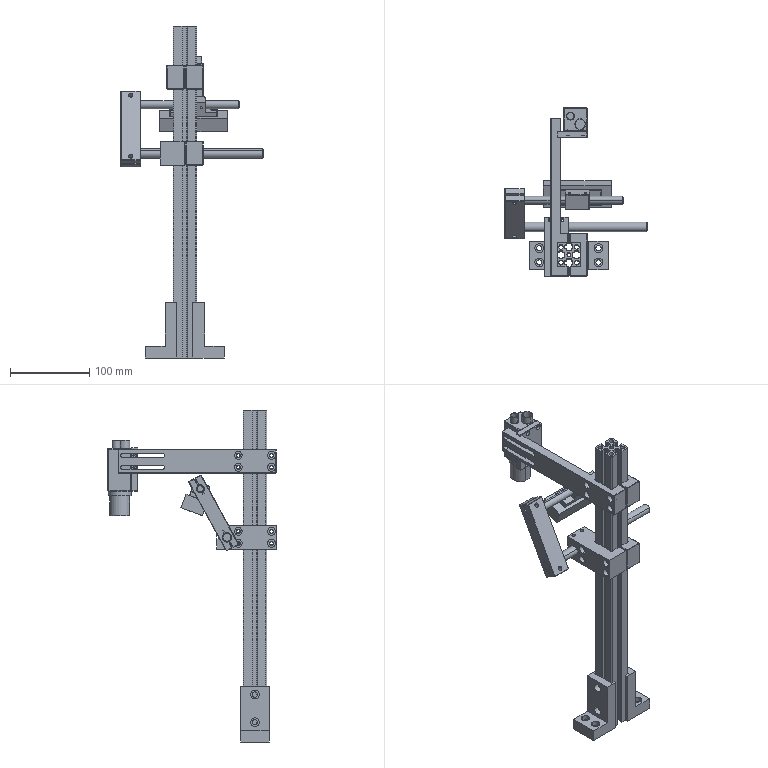Assembly | SolidWorks | mm | 15 component files | 15 solids | 642 faces | box 180 x 213.15 x 420 mm | volume 607746 mm3 | plane 358 | cylinder 256 | cone 16 | spline 12 | commonest cylinder face diameters 1 x48 10 x25 5.5 x24 4.2 x24 6 x20 2 x16 11 x16 6.6 x16
Bill of materials:
connex1100 | 1 |  | Square box-shaped body with rounded vertical edges. Two cylindrical tube stubs stick up from the top face, and a larger cylindrical boss sticks out from the bottom face.
CV-BA-74X27 | 1 |  | Plain rectangular block with two small round holes spaced apart along its length on one face.
TM-50LensCS | 1 |  | Thin-walled hollow cylinder (tube section or ring) that is open at both ends.
XM-WST05-2001 | 1 |  | Long rectangular bar. A rectangular notch near one end leaves two stepped lugs, each with a pair of round holes. The other end has two parallel elongated slots.
XM-WST05-2002 | 1 |  | Rectangular plate with four round holes near the corners and a rectangular notch along one long edge.
XM-WST05-2003 | 1 |  | Base block with two side flanges and a raised central block. The central block has a large through bore. Each flange has a counterbored hole. The central block also has small holes on its side and top faces.
XM-WST05-2004 | 1 |  | Slender solid round rod with small chamfers at both ends.
XM-WST05-2005 | 1 |  | Rectangular block with a rectangular notch on one side. A large round bore runs through the block, and a narrow slot cuts from the bore out to one end face (split-clamp style). There are four holes on the bore face and two holes on the top face.
XM-WST05-2006 | 1 |  | Slender solid round rod with small chamfers at both ends.
XM-WST05-2007 | 1 |  | Long straight extruded bar with a square cross-section. Each side has a central slot with an undercut. Inside there is a central round hole and four larger round holes near the corners. Outer corners are rounded.
XM-WST05-2008 | 2 |  | L-shaped angle bracket with a thick base and an upright. The base has two counterbored holes and the upright has two round holes. A small step runs along one edge of the upright.
XM-WST05-2009 | 2 |  | U-shaped (channel-shaped) block: a rectangular block with a wide rectangular slot cut along its length. One long outer face has four round holes in a rectangular pattern.
XM-WST05-2010 | 1 |  | Elongated rectangular bar/block with a narrow longitudinal slot, two larger circular through-holes on one face that the slot runs through, and two smaller round holes near the ends on the adjacent broad face. Its shape matches a split-clamp style block, but this is an inference.
Mates:
1. concentric | XM-WST05-2005-1 face at (-185.071, 84.169, 359.808) dir (1, 0, 0) r 6 | XM-WST05-2006-1 face at (-235.071, 84.169, 359.808) dir (1, 0, 0) r 6
2. distance | XM-WST05-2005-1 face at (-155.071, 96.669, 374.808) dir (1, 0, 0) | XM-WST05-2006-1 face at (-55.071, 84.169, 359.808) dir (1, 0, 0)
3. coincident | XM-WST05-2005-1 face at (-169.071, 33.669, 374.808) dir (1, 0, 0) | XM-WST05-2007-1 face at (-169.071, 62.669, 100.899) dir (-1, 0, 0)
4. coincident | XM-WST05-2005-1 face at (-169.071, 33.669, 374.808) dir (0, 1, 0) | XM-WST05-2007-1 face at (-157.721, 33.669, 100.899) dir (0, -1, 0)
5. coincident | XM-WST05-2007-1 face at (-139.071, 45.019, 100.899) dir (1, 0, 0) | XM-WST05-2008-1 face at (-139.071, 63.669, 100.899) dir (-1, 0, 0)
6. coincident | XM-WST05-2007-1 face at (-140.071, 33.669, 100.899) dir (0, -1, 0) | XM-WST05-2008-1 face at (-149.071, 33.669, 100.899) dir (0, 1, 0)
7. coincident | XM-WST05-2007-1 face at (-150.421, 63.169, 100.899) dir (0, 0, -1) | XM-WST05-2008-1 face at (-144.071, 30.669, 100.899) dir (0, 0, -1)
8. coincident | XM-WST05-2007-1 face at (-169.071, 45.019, 100.899) dir (-1, 0, 0) | XM-WST05-2008-2 face at (-169.071, 33.669, 100.899) dir (1, 0, 0)
9. coincident | XM-WST05-2008-1 face at (-144.071, 30.669, 100.899) dir (0, 0, -1) | XM-WST05-2008-2 face at (-164.071, 66.669, 100.899) dir (0, 0, -1)
10. coincident | XM-WST05-2007-1 face at (-157.721, 63.669, 100.899) dir (0, 1, 0) | XM-WST05-2008-2 face at (-159.071, 63.669, 100.899) dir (0, -1, 0)
11. coincident | XM-WST05-2007-1 face at (-139.071, 62.669, 100.899) dir (1, 0, 0) | XM-WST05-2009-1 face at (-139.071, 33.669, 344.808) dir (-1, 0, 0)
12. coincident | XM-WST05-2007-1 face at (-140.071, 33.669, 100.899) dir (0, -1, 0) | XM-WST05-2009-1 face at (-167.071, 33.669, 344.808) dir (0, 1, 0)
13. coincident | XM-WST05-2005-1 face at (-185.071, 21.669, 374.808) dir (0, 0, 1) | XM-WST05-2009-1 face at (-153.071, 21.669, 374.808) dir (0, 0, 1)
14. coincident | XM-WST05-2001-1 face at (-155.071, 21.669, 470.899) dir (0, 0, 1) | XM-WST05-2009-3 face at (-153.071, 21.669, 470.899) dir (0, 0, 1)
15. coincident | XM-WST05-2002-1 face at (-169.071, 204.819, 473.399) dir (0, 1, 0) | connex1100-1 face at (-131.071, 204.819, 472.399) dir (0, -1, 0)
16. coincident | XM-WST05-2002-1 face at (-131.071, 204.819, 418.399) dir (1, 0, 0) | connex1100-1 face at (-131.071, 204.819, 472.399) dir (1, 0, 0)
17. distance | XM-WST05-2002-1 face at (-131.071, 204.819, 473.399) dir (0, 0, 1) | connex1100-1 face at (-161.071, 234.819, 472.399) dir (0, 0, 1)
18. concentric | XM-WST05-2006-1 face at (-235.071, 84.169, 359.808) dir (1, 0, 0) r 6 | XM-WST05-2010-1 face at (-210.071, 84.169, 359.808) dir (-1, 0, 0) r 6
19. concentric | XM-WST05-2004-1 face at (-85.071, 117.709, 421.25) dir (-1, 0, 0) r 5 | XM-WST05-2010-1 face at (-210.071, 117.709, 421.25) dir (-1, 0, 0) r 5
20. coincident | XM-WST05-2001-1 face at (-155.071, 63.669, 440.899) dir (0, -1, 0) | XM-WST05-2009-3 face at (-167.071, 63.669, 440.899) dir (0, -1, 0)
21. coincident | XM-WST05-2001-1 face at (-169.071, 63.669, 440.899) dir (1, 0, 0) | XM-WST05-2007-1 face at (-169.071, 62.669, 100.899) dir (-1, 0, 0)
22. coincident | XM-WST05-2001-1 face at (-155.071, 63.669, 440.899) dir (0, -1, 0) | XM-WST05-2007-1 face at (-140.071, 63.669, 100.899) dir (0, 1, 0)
23. coincident | XM-WST05-2007-1 face at (-139.071, 45.019, 100.899) dir (1, 0, 0) | XM-WST05-2009-3 face at (-139.071, 33.669, 440.899) dir (-1, 0, 0)
24. coincident | XM-WST05-2001-1 face at (-165.071, 221.669, 440.899) dir (1, 0, 0) | XM-WST05-2002-1 face at (-165.071, 196.819, 440.899) dir (-1, 0, 0)
25. coincident | XM-WST05-2001-1 face at (-155.071, 21.669, 470.899) dir (0, 0, 1) | XM-WST05-2002-1 face at (-173.071, 196.819, 470.899) dir (0, 0, -1)
26. concentric | connex1100-1 face at (-146.071, 219.819, 412.399) dir (0, 0, 1) r 14.5 | TM-50LensCS-1 face at (-146.071, 219.819, 412.399) dir (0, 0, -1) r 12.7
27. coincident | connex1100-1 face at (-146.071, 219.819, 412.399) dir (0, 0, -1) | TM-50LensCS-1 face at (-146.071, 219.819, 412.399) dir (0, 0, 1)
28. coincident | CV-BA-74X27-1 face at (-143.297, 122.354, 409.108) dir (0, -0.3573, 0.934) | XM-WST05-2003-1 face at (-143.297, 122.354, 409.108) dir (0, 0.3573, -0.934)
29. coincident | CV-BA-74X27-1 plane at (-143.297, 122.354, 409.108) dir (1, 0, 0) | XM-WST05-2003-1 plane at (-143.297, 122.354, 409.108) dir (-1, 0, 0)
30. coincident | CV-BA-74X27-1 plane at (-143.297, 122.354, 409.108) dir (0, -0.934, -0.3573) | XM-WST05-2003-1 plane at (-143.297, 122.354, 409.108) dir (0, -0.934, -0.3573)
31. concentric | XM-WST05-2004-1 face at (-85.071, 117.709, 421.25) dir (-1, 0, 0) r 5 | XM-WST05-2003-1 face at (-113.297, 117.709, 421.25) dir (-1, 0, 0) r 5
32. distance | XM-WST05-2001-1 face at (-155.071, 21.669, 470.899) dir (0, 0, 1) | XM-WST05-2007-1 face at (-150.421, 63.169, 520.899) dir (0, 0, 1)
33. distance | XM-WST05-2001-1 face at (-155.071, 215.669, 463.399) dir (-1, 0, 0) r 2.75 | XM-WST05-2002-1 face at (-165.071, 200.819, 463.399) dir (-1, 0, 0) r 2.1
34. coincident | XM-WST05-2004-1 face at (-235.071, 117.709, 421.25) dir (-1, 0, 0) | XM-WST05-2010-1 face at (-235.071, 116.997, 438.728) dir (-1, 0, 0)
35. coincident | XM-WST05-2006-1 face at (-235.071, 84.169, 359.808) dir (-1, 0, 0) | XM-WST05-2010-1 face at (-235.071, 116.997, 438.728) dir (-1, 0, 0)